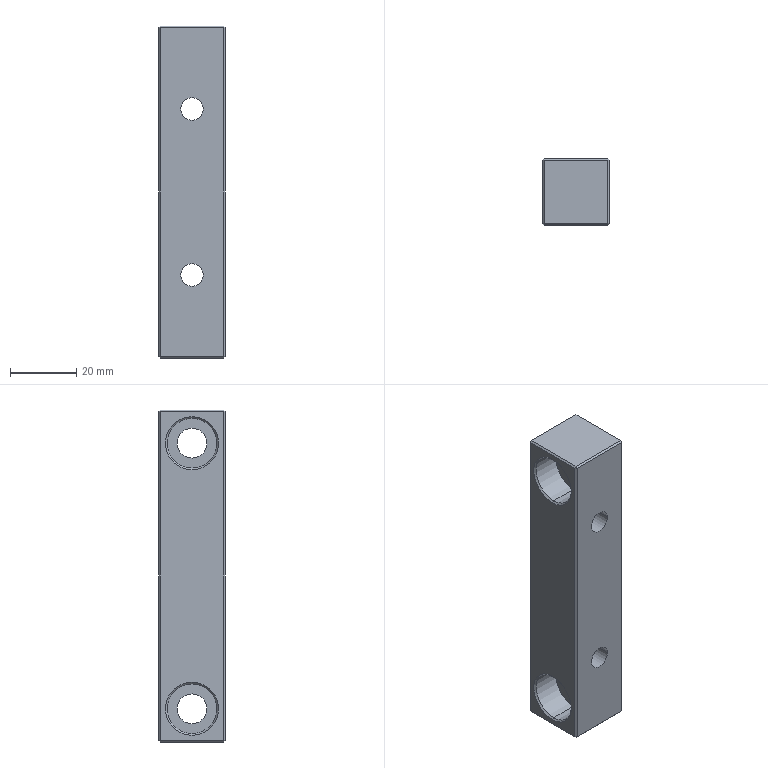Component | SolidWorks | ServoMotorSideFixingPlate-1 | 1 solid | 48 faces | box 20 x 20 x 100 mm | volume 33878 mm3 | plane 28 | cylinder 12 | cone 8 | commonest cylinder face diameters 6.8 x4 15 x4 9 x4 | material 1060 Alloy
build123d program:
from build123d import *

# Parameters (mm, degrees)
SKETCH1_W                                          = 100
SKETCH1_H                                          = 20
BOSS_EXTRUDE1_DEPTH                                = 10
HOLE_SIZE_ACCORDING_TO_TYPE_OF_HEXAGON_D           = 9
HOLE_SIZE_ACCORDING_TO_TYPE_OF_HEXAGON_CBORE_D     = 15
HOLE_SIZE_ACCORDING_TO_TYPE_OF_HEXAGON_CBORE_DEPTH = 9
CHAMFER1_SIZE                                      = 0.5
M8_TAPPED_HOLE1_D                                  = 6.8


with BuildPart() as part:
    # Sketch1 → Boss-Extrude1 (new, symmetric)
    with BuildSketch(Plane.XY):
        Rectangle(SKETCH1_W, SKETCH1_H)
    extrude(amount=BOSS_EXTRUDE1_DEPTH, both=True)

    # Hole Size _according to_ type of Hexagon (through all)
    with Locations(Plane.XY.offset(10)):
        with Locations((-40, 0), (40, 0)):
            CounterBoreHole(HOLE_SIZE_ACCORDING_TO_TYPE_OF_HEXAGON_D / 2, HOLE_SIZE_ACCORDING_TO_TYPE_OF_HEXAGON_CBORE_D / 2, HOLE_SIZE_ACCORDING_TO_TYPE_OF_HEXAGON_CBORE_DEPTH)

    # Chamfer1
    chamfer1_edges = [part.edges().sort_by_distance(p)[0] for p in [
        (50, 0, 10),
        (0, 10, 10),
        (32.5, 0, 10),
        (44.5, 0, -10),
        (-47.5, 0, 10),
        (-35.5, 0, -10),
        (-50, 0, 10),
        (0, 10, -10),
        (50, 0, -10),
        (0, -10, -10),
        (-50, 0, -10),
        (0, -10, 10),
        (-50, 10, 0),
        (50, 10, 0),
        (50, -10, 0),
        (-50, -10, 0),
    ]]
    chamfer(chamfer1_edges, length=CHAMFER1_SIZE)

    # M8 Tapped Hole1 (through all)
    with Locations(Plane(origin=(0, -10, 0), x_dir=(-1, 0, 0), z_dir=(0, -1, 0))):
        with Locations((25, 0), (-25, 0)):
            Hole(M8_TAPPED_HOLE1_D / 2)


solid = part.part

# Placed as in the assembly
solid = solid.moved(Location((25.334, 138.264, 99), (0, -90, 0)))